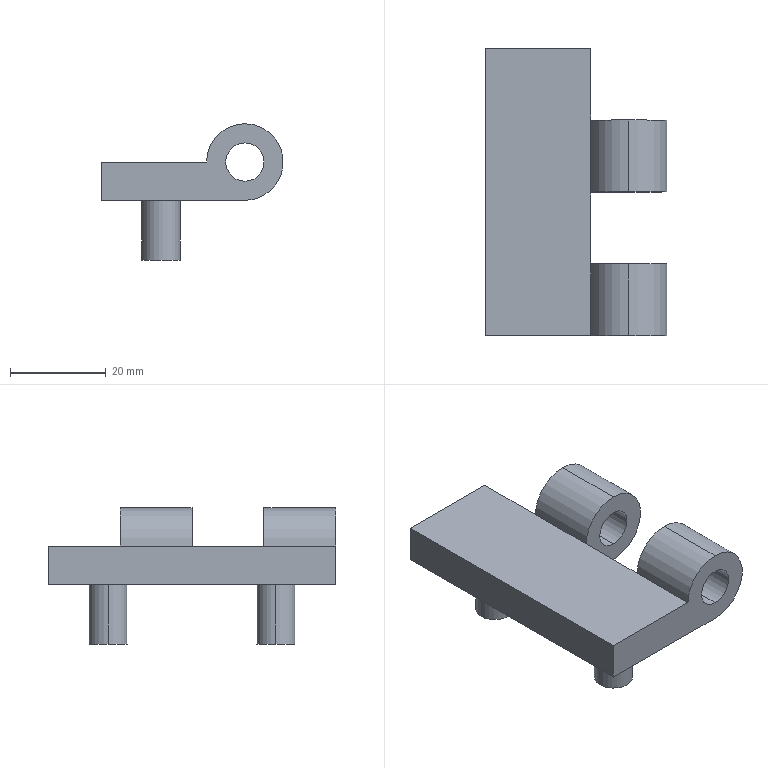Component | SolidWorks | DoorHinge2-2 | 1 solid | 24 faces | box 38 x 60 x 28.5 mm | volume 16753 mm3 | cylinder 12 | plane 12 | commonest cylinder face diameters 8 x8 16 x4
build123d program:
from build123d import *

# Parameters (mm, degrees)
SKETCH2_R           = 8
BOSS_EXTRUDE2_DEPTH = 60
SKETCH3_R           = 4
BOSS_EXTRUDE3_DEPTH = 12.5
SKETCH4_R           = 4
CUT_EXTRUDE1_DEPTH  = 71.144
SKETCH6_W           = 16
SKETCH6_H           = 15
CUT_EXTRUDE3_DEPTH  = 58


with BuildPart() as part:
    # Sketch2 → Boss-Extrude2 (new body)
    with BuildSketch(Plane(origin=(0, 0, 0), x_dir=(1, 0, 0), z_dir=(0, 1, 0))):
        Circle(SKETCH2_R)
        with BuildLine():
            ThreePointArc((8, 0), (5.657, -5.657), (0, -8))
            Line((0, -8), (30, -8))
            Line((30, -8), (30, 0))
            Line((30, 0), (8, 0))
        make_face()
    extrude(amount=BOSS_EXTRUDE2_DEPTH)

    # Sketch3 → Boss-Extrude3 (add)
    with BuildSketch(Plane.XY.offset(8)):
        with Locations(Location((17.5, 47.5, 0), (0, 0, 180))):
            Circle(SKETCH3_R)
        with Locations(Location((17.5, 12.5, 0), (0, 0, 180))):
            Circle(SKETCH3_R)
    extrude(amount=BOSS_EXTRUDE3_DEPTH)

    # Sketch4 → Cut-Extrude1 (cut, through all)
    with BuildSketch(Plane(origin=(0, 60, 0), x_dir=(1, 0, 0), z_dir=(0, 1, 0))):
        with Locations(Location((0, 0, 0), (0, 0, 270))):
            Circle(SKETCH4_R)
    extrude(amount=-CUT_EXTRUDE1_DEPTH, mode=Mode.SUBTRACT)

    # Sketch6 → Cut-Extrude3 (cut)
    with BuildSketch(Plane.XY.offset(8)):
        with Locations((0, 52.5)):
            Rectangle(SKETCH6_W, SKETCH6_H)
        with Locations((0, 22.5)):
            Rectangle(SKETCH6_W, SKETCH6_H)
    extrude(amount=-CUT_EXTRUDE3_DEPTH, mode=Mode.SUBTRACT)


solid = part.part

# Placed as in the assembly
solid = solid.moved(Location((2175.473, 210.46, 1245.107), (-180, 0, 180)))
STEP:
#1=CARTESIAN_POINT('',(85.649,9.467,48.862));
#2=VERTEX_POINT('',#1);
#3=CARTESIAN_POINT('',(85.649,9.467,49.177));
#4=VERTEX_POINT('',#3);
#5=CARTESIAN_POINT('',(85.649,9.467,49.02));
#6=DIRECTION('',(0.,-1.,0.));
#7=DIRECTION('',(0.,0.,-1.));
#8=AXIS2_PLACEMENT_3D('',#5,#6,#7);
#9=CIRCLE('',#8,0.1575);
#10=EDGE_CURVE('',#2,#4,#9,.T.);
#11=ORIENTED_EDGE('',*,*,#10,.T.);
#12=CARTESIAN_POINT('',(85.649,10.057,49.177));
#13=VERTEX_POINT('',#12);
#14=CARTESIAN_POINT('',(85.649,8.286,49.177));
#15=DIRECTION('',(-0.,1.,-0.));
#16=VECTOR('',#15,39.37);
#17=LINE('',#14,#16);
#18=EDGE_CURVE('',#4,#13,#17,.T.);
#19=ORIENTED_EDGE('',*,*,#18,.T.);
#20=CARTESIAN_POINT('',(85.649,10.057,48.862));
#21=VERTEX_POINT('',#20);
#22=CARTESIAN_POINT('',(85.649,10.057,49.02));
#23=DIRECTION('',(-0.,1.,-0.));
#24=DIRECTION('',(0.,0.,1.));
#25=AXIS2_PLACEMENT_3D('',#22,#23,#24);
#26=CIRCLE('',#25,0.1575);
#27=EDGE_CURVE('',#13,#21,#26,.T.);
#28=ORIENTED_EDGE('',*,*,#27,.T.);
#29=CARTESIAN_POINT('',(85.649,8.286,48.862));
#30=DIRECTION('',(-0.,1.,-0.));
#31=VECTOR('',#30,39.37);
#32=LINE('',#29,#31);
#33=EDGE_CURVE('',#2,#21,#32,.T.);
#34=ORIENTED_EDGE('',*,*,#33,.F.);
#35=EDGE_LOOP('',(#11,#19,#28,#34));
#36=FACE_OUTER_BOUND('',#35,.T.);
#37=CARTESIAN_POINT('',(85.649,8.286,49.02));
#38=DIRECTION('',(-0.,1.,-0.));
#39=DIRECTION('',(0.,0.,-1.));
#40=AXIS2_PLACEMENT_3D('',#37,#38,#39);
#41=CYLINDRICAL_SURFACE('',#40,0.1575);
#42=ADVANCED_FACE('',(#36),#41,.F.);
#43=CARTESIAN_POINT('',(84.802,8.778,48.213));
#44=VERTEX_POINT('',#43);
#45=CARTESIAN_POINT('',(85.117,8.778,48.213));
#46=VERTEX_POINT('',#45);
#47=CARTESIAN_POINT('',(84.96,8.778,48.213));
#48=DIRECTION('',(0.,0.,-1.));
#49=DIRECTION('',(-1.,0.,0.));
#50=AXIS2_PLACEMENT_3D('',#47,#48,#49);
#51=CIRCLE('',#50,0.1575);
#52=EDGE_CURVE('',#44,#46,#51,.T.);
#53=ORIENTED_EDGE('',*,*,#52,.F.);
#54=CARTESIAN_POINT('',(84.802,8.778,48.705));
#55=VERTEX_POINT('',#54);
#56=CARTESIAN_POINT('',(84.802,8.778,48.213));
#57=DIRECTION('',(0.,-0.,1.));
#58=VECTOR('',#57,39.37);
#59=LINE('',#56,#58);
#60=EDGE_CURVE('',#44,#55,#59,.T.);
#61=ORIENTED_EDGE('',*,*,#60,.T.);
#62=CARTESIAN_POINT('',(85.117,8.778,48.705));
#63=VERTEX_POINT('',#62);
#64=CARTESIAN_POINT('',(84.96,8.778,48.705));
#65=DIRECTION('',(0.,0.,-1.));
#66=DIRECTION('',(1.,0.,0.));
#67=AXIS2_PLACEMENT_3D('',#64,#65,#66);
#68=CIRCLE('',#67,0.1575);
#69=EDGE_CURVE('',#55,#63,#68,.T.);
#70=ORIENTED_EDGE('',*,*,#69,.T.);
#71=CARTESIAN_POINT('',(85.117,8.778,48.213));
#72=DIRECTION('',(0.,-0.,1.));
#73=VECTOR('',#72,39.37);
#74=LINE('',#71,#73);
#75=EDGE_CURVE('',#46,#63,#74,.T.);
#76=ORIENTED_EDGE('',*,*,#75,.F.);
#77=EDGE_LOOP('',(#53,#61,#70,#76));
#78=FACE_OUTER_BOUND('',#77,.T.);
#79=CARTESIAN_POINT('',(84.96,8.778,48.213));
#80=DIRECTION('',(0.,-0.,1.));
#81=DIRECTION('',(1.,0.,0.));
#82=AXIS2_PLACEMENT_3D('',#79,#80,#81);
#83=CYLINDRICAL_SURFACE('',#82,0.1575);
#84=ADVANCED_FACE('',(#78),#83,.T.);
#85=CARTESIAN_POINT('',(84.802,10.156,48.213));
#86=VERTEX_POINT('',#85);
#87=CARTESIAN_POINT('',(85.117,10.156,48.213));
#88=VERTEX_POINT('',#87);
#89=CARTESIAN_POINT('',(84.96,10.156,48.213));
#90=DIRECTION('',(0.,0.,-1.));
#91=DIRECTION('',(-1.,0.,0.));
#92=AXIS2_PLACEMENT_3D('',#89,#90,#91);
#93=CIRCLE('',#92,0.1575);
#94=EDGE_CURVE('',#86,#88,#93,.T.);
#95=ORIENTED_EDGE('',*,*,#94,.F.);
#96=CARTESIAN_POINT('',(84.802,10.156,48.705));
#97=VERTEX_POINT('',#96);
#98=CARTESIAN_POINT('',(84.802,10.156,48.213));
#99=DIRECTION('',(0.,-0.,1.));
#100=VECTOR('',#99,39.37);
#101=LINE('',#98,#100);
#102=EDGE_CURVE('',#86,#97,#101,.T.);
#103=ORIENTED_EDGE('',*,*,#102,.T.);
#104=CARTESIAN_POINT('',(85.117,10.156,48.705));
#105=VERTEX_POINT('',#104);
#106=CARTESIAN_POINT('',(84.96,10.156,48.705));
#107=DIRECTION('',(0.,0.,-1.));
#108=DIRECTION('',(1.,0.,0.));
#109=AXIS2_PLACEMENT_3D('',#106,#107,#108);
#110=CIRCLE('',#109,0.1575);
#111=EDGE_CURVE('',#97,#105,#110,.T.);
#112=ORIENTED_EDGE('',*,*,#111,.T.);
#113=CARTESIAN_POINT('',(85.117,10.156,48.213));
#114=DIRECTION('',(0.,-0.,1.));
#115=VECTOR('',#114,39.37);
#116=LINE('',#113,#115);
#117=EDGE_CURVE('',#88,#105,#116,.T.);
#118=ORIENTED_EDGE('',*,*,#117,.F.);
#119=EDGE_LOOP('',(#95,#103,#112,#118));
#120=FACE_OUTER_BOUND('',#119,.T.);
#121=CARTESIAN_POINT('',(84.96,10.156,48.213));
#122=DIRECTION('',(0.,-0.,1.));
#123=DIRECTION('',(1.,0.,0.));
#124=AXIS2_PLACEMENT_3D('',#121,#122,#123);
#125=CYLINDRICAL_SURFACE('',#124,0.1575);
#126=ADVANCED_FACE('',(#120),#125,.T.);
#127=CARTESIAN_POINT('',(85.649,10.057,48.705));
#128=VERTEX_POINT('',#127);
#129=CARTESIAN_POINT('',(85.649,10.057,49.335));
#130=VERTEX_POINT('',#129);
#131=CARTESIAN_POINT('',(85.649,10.057,49.02));
#132=DIRECTION('',(0.,-1.,0.));
#133=DIRECTION('',(0.,0.,1.));
#134=AXIS2_PLACEMENT_3D('',#131,#132,#133);
#135=CIRCLE('',#134,0.315);
#136=EDGE_CURVE('',#128,#130,#135,.T.);
#137=ORIENTED_EDGE('',*,*,#136,.T.);
#138=CARTESIAN_POINT('',(85.649,9.467,49.335));
#139=VERTEX_POINT('',#138);
#140=CARTESIAN_POINT('',(85.649,10.648,49.335));
#141=DIRECTION('',(0.,-1.,0.));
#142=VECTOR('',#141,39.37);
#143=LINE('',#140,#142);
#144=EDGE_CURVE('',#130,#139,#143,.T.);
#145=ORIENTED_EDGE('',*,*,#144,.T.);
#146=CARTESIAN_POINT('',(85.649,9.467,48.705));
#147=VERTEX_POINT('',#146);
#148=CARTESIAN_POINT('',(85.649,9.467,49.02));
#149=DIRECTION('',(-0.,1.,-0.));
#150=DIRECTION('',(0.,0.,-1.));
#151=AXIS2_PLACEMENT_3D('',#148,#149,#150);
#152=CIRCLE('',#151,0.315);
#153=EDGE_CURVE('',#139,#147,#152,.T.);
#154=ORIENTED_EDGE('',*,*,#153,.T.);
#155=CARTESIAN_POINT('',(85.649,10.648,48.705));
#156=DIRECTION('',(0.,-1.,0.));
#157=VECTOR('',#156,39.37);
#158=LINE('',#155,#157);
#159=EDGE_CURVE('',#128,#147,#158,.T.);
#160=ORIENTED_EDGE('',*,*,#159,.F.);
#161=EDGE_LOOP('',(#137,#145,#154,#160));
#162=FACE_OUTER_BOUND('',#161,.T.);
#163=CARTESIAN_POINT('',(85.649,10.648,49.02));
#164=DIRECTION('',(0.,-1.,0.));
#165=DIRECTION('',(0.,0.,1.));
#166=AXIS2_PLACEMENT_3D('',#163,#164,#165);
#167=CYLINDRICAL_SURFACE('',#166,0.315);
#168=ADVANCED_FACE('',(#162),#167,.T.);
#169=CARTESIAN_POINT('',(85.649,8.286,49.177));
#170=VERTEX_POINT('',#169);
#171=CARTESIAN_POINT('',(85.649,8.286,48.862));
#172=VERTEX_POINT('',#171);
#173=CARTESIAN_POINT('',(85.649,8.286,49.02));
#174=DIRECTION('',(-0.,1.,-0.));
#175=DIRECTION('',(0.,0.,-1.));
#176=AXIS2_PLACEMENT_3D('',#173,#174,#175);
#177=CIRCLE('',#176,0.1575);
#178=EDGE_CURVE('',#170,#172,#177,.T.);
#179=ORIENTED_EDGE('',*,*,#178,.F.);
#180=CARTESIAN_POINT('',(85.649,8.876,49.177));
#181=VERTEX_POINT('',#180);
#182=CARTESIAN_POINT('',(85.649,8.286,49.177));
#183=DIRECTION('',(-0.,1.,-0.));
#184=VECTOR('',#183,39.37);
#185=LINE('',#182,#184);
#186=EDGE_CURVE('',#170,#181,#185,.T.);
#187=ORIENTED_EDGE('',*,*,#186,.T.);
#188=CARTESIAN_POINT('',(85.649,8.876,48.862));
#189=VERTEX_POINT('',#188);
#190=CARTESIAN_POINT('',(85.649,8.876,49.02));
#191=DIRECTION('',(0.,1.,-0.));
#192=DIRECTION('',(-1.,0.,0.));
#193=AXIS2_PLACEMENT_3D('',#190,#191,#192);
#194=CIRCLE('',#193,0.1575);
#195=EDGE_CURVE('',#181,#189,#194,.T.);
#196=ORIENTED_EDGE('',*,*,#195,.T.);
#197=CARTESIAN_POINT('',(85.649,8.286,48.862));
#198=DIRECTION('',(-0.,1.,-0.));
#199=VECTOR('',#198,39.37);
#200=LINE('',#197,#199);
#201=EDGE_CURVE('',#172,#189,#200,.T.);
#202=ORIENTED_EDGE('',*,*,#201,.F.);
#203=EDGE_LOOP('',(#179,#187,#196,#202));
#204=FACE_OUTER_BOUND('',#203,.T.);
#205=CARTESIAN_POINT('',(85.649,8.286,49.02));
#206=DIRECTION('',(-0.,1.,-0.));
#207=DIRECTION('',(0.,0.,-1.));
#208=AXIS2_PLACEMENT_3D('',#205,#206,#207);
#209=CYLINDRICAL_SURFACE('',#208,0.1575);
#210=ADVANCED_FACE('',(#204),#209,.F.);
#211=CARTESIAN_POINT('',(85.649,8.876,48.705));
#212=VERTEX_POINT('',#211);
#213=CARTESIAN_POINT('',(85.649,8.876,49.335));
#214=VERTEX_POINT('',#213);
#215=CARTESIAN_POINT('',(85.649,8.876,49.02));
#216=DIRECTION('',(-0.,-1.,0.));
#217=DIRECTION('',(-1.,0.,0.));
#218=AXIS2_PLACEMENT_3D('',#215,#216,#217);
#219=CIRCLE('',#218,0.315);
#220=EDGE_CURVE('',#212,#214,#219,.T.);
#221=ORIENTED_EDGE('',*,*,#220,.T.);
#222=CARTESIAN_POINT('',(85.649,8.286,49.335));
#223=VERTEX_POINT('',#222);
#224=CARTESIAN_POINT('',(85.649,10.648,49.335));
#225=DIRECTION('',(0.,-1.,0.));
#226=VECTOR('',#225,39.37);
#227=LINE('',#224,#226);
#228=EDGE_CURVE('',#214,#223,#227,.T.);
#229=ORIENTED_EDGE('',*,*,#228,.T.);
#230=CARTESIAN_POINT('',(85.649,8.286,48.705));
#231=VERTEX_POINT('',#230);
#232=CARTESIAN_POINT('',(85.649,8.286,49.02));
#233=DIRECTION('',(-0.,1.,-0.));
#234=DIRECTION('',(0.,0.,-1.));
#235=AXIS2_PLACEMENT_3D('',#232,#233,#234);
#236=CIRCLE('',#235,0.315);
#237=EDGE_CURVE('',#223,#231,#236,.T.);
#238=ORIENTED_EDGE('',*,*,#237,.T.);
#239=CARTESIAN_POINT('',(85.649,10.648,48.705));
#240=DIRECTION('',(0.,-1.,0.));
#241=VECTOR('',#240,39.37);
#242=LINE('',#239,#241);
#243=EDGE_CURVE('',#212,#231,#242,.T.);
#244=ORIENTED_EDGE('',*,*,#243,.F.);
#245=EDGE_LOOP('',(#221,#229,#238,#244));
#246=FACE_OUTER_BOUND('',#245,.T.);
#247=CARTESIAN_POINT('',(85.649,10.648,49.02));
#248=DIRECTION('',(0.,-1.,0.));
#249=DIRECTION('',(0.,0.,1.));
#250=AXIS2_PLACEMENT_3D('',#247,#248,#249);
#251=CYLINDRICAL_SURFACE('',#250,0.315);
#252=ADVANCED_FACE('',(#246),#251,.T.);
#253=ORIENTED_EDGE('',*,*,#228,.F.);
#254=CARTESIAN_POINT('',(85.334,8.876,49.02));
#255=VERTEX_POINT('',#254);
#256=CARTESIAN_POINT('',(85.649,8.876,49.02));
#257=DIRECTION('',(-0.,-1.,0.));
#258=DIRECTION('',(-1.,0.,0.));
#259=AXIS2_PLACEMENT_3D('',#256,#257,#258);
#260=CIRCLE('',#259,0.315);
#261=EDGE_CURVE('',#214,#255,#260,.T.);
#262=ORIENTED_EDGE('',*,*,#261,.T.);
#263=CARTESIAN_POINT('',(85.334,8.286,49.02));
#264=VERTEX_POINT('',#263);
#265=CARTESIAN_POINT('',(85.334,10.648,49.02));
#266=DIRECTION('',(0.,-1.,0.));
#267=VECTOR('',#266,39.37);
#268=LINE('',#265,#267);
#269=EDGE_CURVE('',#255,#264,#268,.T.);
#270=ORIENTED_EDGE('',*,*,#269,.T.);
#271=CARTESIAN_POINT('',(85.649,8.286,49.02));
#272=DIRECTION('',(-0.,1.,-0.));
#273=DIRECTION('',(0.,0.,-1.));
#274=AXIS2_PLACEMENT_3D('',#271,#272,#273);
#275=CIRCLE('',#274,0.315);
#276=EDGE_CURVE('',#264,#223,#275,.T.);
#277=ORIENTED_EDGE('',*,*,#276,.T.);
#278=EDGE_LOOP('',(#253,#262,#270,#277));
#279=FACE_OUTER_BOUND('',#278,.T.);
#280=CARTESIAN_POINT('',(85.649,10.648,49.02));
#281=DIRECTION('',(0.,-1.,0.));
#282=DIRECTION('',(0.,0.,1.));
#283=AXIS2_PLACEMENT_3D('',#280,#281,#282);
#284=CYLINDRICAL_SURFACE('',#283,0.315);
#285=ADVANCED_FACE('',(#279),#284,.T.);
#286=ORIENTED_EDGE('',*,*,#186,.F.);
#287=CARTESIAN_POINT('',(85.649,8.286,49.02));
#288=DIRECTION('',(-0.,1.,-0.));
#289=DIRECTION('',(0.,0.,-1.));
#290=AXIS2_PLACEMENT_3D('',#287,#288,#289);
#291=CIRCLE('',#290,0.1575);
#292=EDGE_CURVE('',#172,#170,#291,.T.);
#293=ORIENTED_EDGE('',*,*,#292,.F.);
#294=ORIENTED_EDGE('',*,*,#201,.T.);
#295=CARTESIAN_POINT('',(85.649,8.876,49.02));
#296=DIRECTION('',(0.,1.,-0.));
#297=DIRECTION('',(-1.,0.,0.));
#298=AXIS2_PLACEMENT_3D('',#295,#296,#297);
#299=CIRCLE('',#298,0.1575);
#300=EDGE_CURVE('',#189,#181,#299,.T.);
#301=ORIENTED_EDGE('',*,*,#300,.T.);
#302=EDGE_LOOP('',(#286,#293,#294,#301));
#303=FACE_OUTER_BOUND('',#302,.T.);
#304=CARTESIAN_POINT('',(85.649,8.286,49.02));
#305=DIRECTION('',(-0.,1.,-0.));
#306=DIRECTION('',(0.,0.,-1.));
#307=AXIS2_PLACEMENT_3D('',#304,#305,#306);
#308=CYLINDRICAL_SURFACE('',#307,0.1575);
#309=ADVANCED_FACE('',(#303),#308,.F.);
#310=CARTESIAN_POINT('',(84.96,10.156,48.705));
#311=DIRECTION('',(0.,0.,-1.));
#312=DIRECTION('',(1.,0.,0.));
#313=AXIS2_PLACEMENT_3D('',#310,#311,#312);
#314=CIRCLE('',#313,0.1575);
#315=EDGE_CURVE('',#105,#97,#314,.T.);
#316=ORIENTED_EDGE('',*,*,#315,.F.);
#317=ORIENTED_EDGE('',*,*,#111,.F.);
#318=EDGE_LOOP('',(#316,#317));
#319=FACE_BOUND('',#318,.T.);
#320=CARTESIAN_POINT('',(85.334,8.876,48.705));
#321=VERTEX_POINT('',#320);
#322=CARTESIAN_POINT('',(85.334,9.467,48.705));
#323=VERTEX_POINT('',#322);
#324=CARTESIAN_POINT('',(85.334,8.876,48.705));
#325=DIRECTION('',(0.,1.,-0.));
#326=VECTOR('',#325,39.37);
#327=LINE('',#324,#326);
#328=EDGE_CURVE('',#321,#323,#327,.T.);
#329=ORIENTED_EDGE('',*,*,#328,.F.);
#330=CARTESIAN_POINT('',(85.334,8.876,48.705));
#331=DIRECTION('',(-1.,0.,-0.));
#332=VECTOR('',#331,39.37);
#333=LINE('',#330,#332);
#334=EDGE_CURVE('',#212,#321,#333,.T.);
#335=ORIENTED_EDGE('',*,*,#334,.F.);
#336=ORIENTED_EDGE('',*,*,#243,.T.);
#337=CARTESIAN_POINT('',(84.467,8.286,48.705));
#338=VERTEX_POINT('',#337);
#339=CARTESIAN_POINT('',(86.484,8.286,48.705));
#340=DIRECTION('',(-1.,0.,0.));
#341=VECTOR('',#340,39.37);
#342=LINE('',#339,#341);
#343=EDGE_CURVE('',#231,#338,#342,.T.);
#344=ORIENTED_EDGE('',*,*,#343,.T.);
#345=CARTESIAN_POINT('',(84.467,10.648,48.705));
#346=VERTEX_POINT('',#345);
#347=CARTESIAN_POINT('',(84.467,10.648,48.705));
#348=DIRECTION('',(0.,-1.,0.));
#349=VECTOR('',#348,39.37);
#350=LINE('',#347,#349);
#351=EDGE_CURVE('',#346,#338,#350,.T.);
#352=ORIENTED_EDGE('',*,*,#351,.F.);
#353=CARTESIAN_POINT('',(85.334,10.648,48.705));
#354=VERTEX_POINT('',#353);
#355=CARTESIAN_POINT('',(86.484,10.648,48.705));
#356=DIRECTION('',(-1.,0.,0.));
#357=VECTOR('',#356,39.37);
#358=LINE('',#355,#357);
#359=EDGE_CURVE('',#354,#346,#358,.T.);
#360=ORIENTED_EDGE('',*,*,#359,.F.);
#361=CARTESIAN_POINT('',(85.334,10.057,48.705));
#362=VERTEX_POINT('',#361);
#363=CARTESIAN_POINT('',(85.334,10.057,48.705));
#364=DIRECTION('',(0.,1.,-0.));
#365=VECTOR('',#364,39.37);
#366=LINE('',#363,#365);
#367=EDGE_CURVE('',#362,#354,#366,.T.);
#368=ORIENTED_EDGE('',*,*,#367,.F.);
#369=CARTESIAN_POINT('',(85.334,10.057,48.705));
#370=DIRECTION('',(-1.,0.,0.));
#371=VECTOR('',#370,39.37);
#372=LINE('',#369,#371);
#373=EDGE_CURVE('',#128,#362,#372,.T.);
#374=ORIENTED_EDGE('',*,*,#373,.F.);
#375=ORIENTED_EDGE('',*,*,#159,.T.);
#376=CARTESIAN_POINT('',(85.334,9.467,48.705));
#377=DIRECTION('',(1.,0.,0.));
#378=VECTOR('',#377,39.37);
#379=LINE('',#376,#378);
#380=EDGE_CURVE('',#323,#147,#379,.T.);
#381=ORIENTED_EDGE('',*,*,#380,.F.);
#382=EDGE_LOOP('',(#329,#335,#336,#344,#352,#360,#368,#374,#375,#381));
#383=FACE_OUTER_BOUND('',#382,.T.);
#384=CARTESIAN_POINT('',(84.96,8.778,48.705));
#385=DIRECTION('',(0.,0.,-1.));
#386=DIRECTION('',(1.,0.,0.));
#387=AXIS2_PLACEMENT_3D('',#384,#385,#386);
#388=CIRCLE('',#387,0.1575);
#389=EDGE_CURVE('',#63,#55,#388,.T.);
#390=ORIENTED_EDGE('',*,*,#389,.F.);
#391=ORIENTED_EDGE('',*,*,#69,.F.);
#392=EDGE_LOOP('',(#390,#391));
#393=FACE_BOUND('',#392,.T.);
#394=CARTESIAN_POINT('',(86.484,10.648,48.705));
#395=DIRECTION('',(0.,-0.,1.));
#396=DIRECTION('',(1.,0.,0.));
#397=AXIS2_PLACEMENT_3D('',#394,#395,#396);
#398=PLANE('',#397);
#399=ADVANCED_FACE('',(#319,#383,#393),#398,.F.);
#400=ORIENTED_EDGE('',*,*,#144,.F.);
#401=CARTESIAN_POINT('',(85.334,10.057,49.02));
#402=VERTEX_POINT('',#401);
#403=CARTESIAN_POINT('',(85.649,10.057,49.02));
#404=DIRECTION('',(0.,-1.,0.));
#405=DIRECTION('',(0.,0.,1.));
#406=AXIS2_PLACEMENT_3D('',#403,#404,#405);
#407=CIRCLE('',#406,0.315);
#408=EDGE_CURVE('',#130,#402,#407,.T.);
#409=ORIENTED_EDGE('',*,*,#408,.T.);
#410=CARTESIAN_POINT('',(85.334,9.467,49.02));
#411=VERTEX_POINT('',#410);
#412=CARTESIAN_POINT('',(85.334,10.648,49.02));
#413=DIRECTION('',(0.,-1.,0.));
#414=VECTOR('',#413,39.37);
#415=LINE('',#412,#414);
#416=EDGE_CURVE('',#402,#411,#415,.T.);
#417=ORIENTED_EDGE('',*,*,#416,.T.);
#418=CARTESIAN_POINT('',(85.649,9.467,49.02));
#419=DIRECTION('',(-0.,1.,-0.));
#420=DIRECTION('',(0.,0.,-1.));
#421=AXIS2_PLACEMENT_3D('',#418,#419,#420);
#422=CIRCLE('',#421,0.315);
#423=EDGE_CURVE('',#411,#139,#422,.T.);
#424=ORIENTED_EDGE('',*,*,#423,.T.);
#425=EDGE_LOOP('',(#400,#409,#417,#424));
#426=FACE_OUTER_BOUND('',#425,.T.);
#427=CARTESIAN_POINT('',(85.649,10.648,49.02));
#428=DIRECTION('',(0.,-1.,0.));
#429=DIRECTION('',(0.,0.,1.));
#430=AXIS2_PLACEMENT_3D('',#427,#428,#429);
#431=CYLINDRICAL_SURFACE('',#430,0.315);
#432=ADVANCED_FACE('',(#426),#431,.T.);
#433=CARTESIAN_POINT('',(84.467,8.286,49.02));
#434=VERTEX_POINT('',#433);
#435=CARTESIAN_POINT('',(84.467,8.286,49.02));
#436=DIRECTION('',(0.,-0.,1.));
#437=VECTOR('',#436,39.37);
#438=LINE('',#435,#437);
#439=EDGE_CURVE('',#338,#434,#438,.T.);
#440=ORIENTED_EDGE('',*,*,#439,.T.);
#441=CARTESIAN_POINT('',(84.467,10.648,49.02));
#442=VERTEX_POINT('',#441);
#443=CARTESIAN_POINT('',(84.467,10.648,49.02));
#444=DIRECTION('',(0.,-1.,0.));
#445=VECTOR('',#444,39.37);
#446=LINE('',#443,#445);
#447=EDGE_CURVE('',#442,#434,#446,.T.);
#448=ORIENTED_EDGE('',*,*,#447,.F.);
#449=CARTESIAN_POINT('',(84.467,10.648,49.02));
#450=DIRECTION('',(0.,-0.,1.));
#451=VECTOR('',#450,39.37);
#452=LINE('',#449,#451);
#453=EDGE_CURVE('',#346,#442,#452,.T.);
#454=ORIENTED_EDGE('',*,*,#453,.F.);
#455=ORIENTED_EDGE('',*,*,#351,.T.);
#456=EDGE_LOOP('',(#440,#448,#454,#455));
#457=FACE_OUTER_BOUND('',#456,.T.);
#458=CARTESIAN_POINT('',(84.467,10.648,49.02));
#459=DIRECTION('',(1.,0.,0.));
#460=DIRECTION('',(0.,0.,-1.));
#461=AXIS2_PLACEMENT_3D('',#458,#459,#460);
#462=PLANE('',#461);
#463=ADVANCED_FACE('',(#457),#462,.F.);
#464=CARTESIAN_POINT('',(86.484,8.286,49.02));
#465=DIRECTION('',(1.,-0.,0.));
#466=VECTOR('',#465,39.37);
#467=LINE('',#464,#466);
#468=EDGE_CURVE('',#434,#264,#467,.T.);
#469=ORIENTED_EDGE('',*,*,#468,.T.);
#470=ORIENTED_EDGE('',*,*,#269,.F.);
#471=CARTESIAN_POINT('',(85.334,10.648,49.02));
#472=DIRECTION('',(0.,-1.,0.));
#473=VECTOR('',#472,39.37);
#474=LINE('',#471,#473);
#475=EDGE_CURVE('',#411,#255,#474,.T.);
#476=ORIENTED_EDGE('',*,*,#475,.F.);
#477=ORIENTED_EDGE('',*,*,#416,.F.);
#478=CARTESIAN_POINT('',(85.334,10.648,49.02));
#479=VERTEX_POINT('',#478);
#480=CARTESIAN_POINT('',(85.334,10.648,49.02));
#481=DIRECTION('',(0.,-1.,0.));
#482=VECTOR('',#481,39.37);
#483=LINE('',#480,#482);
#484=EDGE_CURVE('',#479,#402,#483,.T.);
#485=ORIENTED_EDGE('',*,*,#484,.F.);
#486=CARTESIAN_POINT('',(86.484,10.648,49.02));
#487=DIRECTION('',(1.,-0.,0.));
#488=VECTOR('',#487,39.37);
#489=LINE('',#486,#488);
#490=EDGE_CURVE('',#442,#479,#489,.T.);
#491=ORIENTED_EDGE('',*,*,#490,.F.);
#492=ORIENTED_EDGE('',*,*,#447,.T.);
#493=EDGE_LOOP('',(#469,#470,#476,#477,#485,#491,#492));
#494=FACE_OUTER_BOUND('',#493,.T.);
#495=CARTESIAN_POINT('',(86.484,10.648,49.02));
#496=DIRECTION('',(0.,0.,-1.));
#497=DIRECTION('',(-1.,0.,-0.));
#498=AXIS2_PLACEMENT_3D('',#495,#496,#497);
#499=PLANE('',#498);
#500=ADVANCED_FACE('',(#494),#499,.F.);
#501=CARTESIAN_POINT('',(85.334,10.648,50.988));
#502=DIRECTION('',(0.,0.,-1.));
#503=VECTOR('',#502,39.37);
#504=LINE('',#501,#503);
#505=EDGE_CURVE('',#479,#354,#504,.T.);
#506=ORIENTED_EDGE('',*,*,#505,.T.);
#507=ORIENTED_EDGE('',*,*,#359,.T.);
#508=ORIENTED_EDGE('',*,*,#453,.T.);
#509=ORIENTED_EDGE('',*,*,#490,.T.);
#510=EDGE_LOOP('',(#506,#507,#508,#509));
#511=FACE_OUTER_BOUND('',#510,.T.);
#512=CARTESIAN_POINT('',(86.484,10.648,49.02));
#513=DIRECTION('',(-0.,1.,0.));
#514=DIRECTION('',(0.,0.,-1.));
#515=AXIS2_PLACEMENT_3D('',#512,#513,#514);
#516=PLANE('',#515);
#517=ADVANCED_FACE('',(#511),#516,.T.);
#518=ORIENTED_EDGE('',*,*,#292,.T.);
#519=ORIENTED_EDGE('',*,*,#178,.T.);
#520=EDGE_LOOP('',(#518,#519));
#521=FACE_BOUND('',#520,.T.);
#522=ORIENTED_EDGE('',*,*,#276,.F.);
#523=ORIENTED_EDGE('',*,*,#468,.F.);
#524=ORIENTED_EDGE('',*,*,#439,.F.);
#525=ORIENTED_EDGE('',*,*,#343,.F.);
#526=ORIENTED_EDGE('',*,*,#237,.F.);
#527=EDGE_LOOP('',(#522,#523,#524,#525,#526));
#528=FACE_OUTER_BOUND('',#527,.T.);
#529=CARTESIAN_POINT('',(86.484,8.286,49.02));
#530=DIRECTION('',(-0.,1.,0.));
#531=DIRECTION('',(0.,0.,-1.));
#532=AXIS2_PLACEMENT_3D('',#529,#530,#531);
#533=PLANE('',#532);
#534=ADVANCED_FACE('',(#521,#528),#533,.F.);
#535=ORIENTED_EDGE('',*,*,#102,.F.);
#536=CARTESIAN_POINT('',(84.96,10.156,48.213));
#537=DIRECTION('',(0.,0.,-1.));
#538=DIRECTION('',(-1.,0.,0.));
#539=AXIS2_PLACEMENT_3D('',#536,#537,#538);
#540=CIRCLE('',#539,0.1575);
#541=EDGE_CURVE('',#88,#86,#540,.T.);
#542=ORIENTED_EDGE('',*,*,#541,.F.);
#543=ORIENTED_EDGE('',*,*,#117,.T.);
#544=ORIENTED_EDGE('',*,*,#315,.T.);
#545=EDGE_LOOP('',(#535,#542,#543,#544));
#546=FACE_OUTER_BOUND('',#545,.T.);
#547=CARTESIAN_POINT('',(84.96,10.156,48.213));
#548=DIRECTION('',(0.,-0.,1.));
#549=DIRECTION('',(1.,0.,0.));
#550=AXIS2_PLACEMENT_3D('',#547,#548,#549);
#551=CYLINDRICAL_SURFACE('',#550,0.1575);
#552=ADVANCED_FACE('',(#546),#551,.T.);
#553=ORIENTED_EDGE('',*,*,#541,.T.);
#554=ORIENTED_EDGE('',*,*,#94,.T.);
#555=EDGE_LOOP('',(#553,#554));
#556=FACE_OUTER_BOUND('',#555,.T.);
#557=CARTESIAN_POINT('',(84.96,10.156,48.213));
#558=DIRECTION('',(0.,0.,-1.));
#559=DIRECTION('',(-1.,0.,0.));
#560=AXIS2_PLACEMENT_3D('',#557,#558,#559);
#561=PLANE('',#560);
#562=ADVANCED_FACE('',(#556),#561,.T.);
#563=ORIENTED_EDGE('',*,*,#60,.F.);
#564=CARTESIAN_POINT('',(84.96,8.778,48.213));
#565=DIRECTION('',(0.,0.,-1.));
#566=DIRECTION('',(-1.,0.,0.));
#567=AXIS2_PLACEMENT_3D('',#564,#565,#566);
#568=CIRCLE('',#567,0.1575);
#569=EDGE_CURVE('',#46,#44,#568,.T.);
#570=ORIENTED_EDGE('',*,*,#569,.F.);
#571=ORIENTED_EDGE('',*,*,#75,.T.);
#572=ORIENTED_EDGE('',*,*,#389,.T.);
#573=EDGE_LOOP('',(#563,#570,#571,#572));
#574=FACE_OUTER_BOUND('',#573,.T.);
#575=CARTESIAN_POINT('',(84.96,8.778,48.213));
#576=DIRECTION('',(0.,-0.,1.));
#577=DIRECTION('',(1.,0.,0.));
#578=AXIS2_PLACEMENT_3D('',#575,#576,#577);
#579=CYLINDRICAL_SURFACE('',#578,0.1575);
#580=ADVANCED_FACE('',(#574),#579,.T.);
#581=ORIENTED_EDGE('',*,*,#569,.T.);
#582=ORIENTED_EDGE('',*,*,#52,.T.);
#583=EDGE_LOOP('',(#581,#582));
#584=FACE_OUTER_BOUND('',#583,.T.);
#585=CARTESIAN_POINT('',(84.96,8.778,48.213));
#586=DIRECTION('',(0.,0.,-1.));
#587=DIRECTION('',(-1.,0.,0.));
#588=AXIS2_PLACEMENT_3D('',#585,#586,#587);
#589=PLANE('',#588);
#590=ADVANCED_FACE('',(#584),#589,.T.);
#591=ORIENTED_EDGE('',*,*,#18,.F.);
#592=CARTESIAN_POINT('',(85.649,9.467,49.02));
#593=DIRECTION('',(0.,-1.,0.));
#594=DIRECTION('',(0.,0.,-1.));
#595=AXIS2_PLACEMENT_3D('',#592,#593,#594);
#596=CIRCLE('',#595,0.1575);
#597=EDGE_CURVE('',#4,#2,#596,.T.);
#598=ORIENTED_EDGE('',*,*,#597,.T.);
#599=ORIENTED_EDGE('',*,*,#33,.T.);
#600=CARTESIAN_POINT('',(85.649,10.057,49.02));
#601=DIRECTION('',(-0.,1.,-0.));
#602=DIRECTION('',(0.,0.,1.));
#603=AXIS2_PLACEMENT_3D('',#600,#601,#602);
#604=CIRCLE('',#603,0.1575);
#605=EDGE_CURVE('',#21,#13,#604,.T.);
#606=ORIENTED_EDGE('',*,*,#605,.T.);
#607=EDGE_LOOP('',(#591,#598,#599,#606));
#608=FACE_OUTER_BOUND('',#607,.T.);
#609=CARTESIAN_POINT('',(85.649,8.286,49.02));
#610=DIRECTION('',(-0.,1.,-0.));
#611=DIRECTION('',(0.,0.,-1.));
#612=AXIS2_PLACEMENT_3D('',#609,#610,#611);
#613=CYLINDRICAL_SURFACE('',#612,0.1575);
#614=ADVANCED_FACE('',(#608),#613,.F.);
#615=CARTESIAN_POINT('',(85.334,10.057,50.988));
#616=DIRECTION('',(0.,0.,-1.));
#617=VECTOR('',#616,39.37);
#618=LINE('',#615,#617);
#619=EDGE_CURVE('',#402,#362,#618,.T.);
#620=ORIENTED_EDGE('',*,*,#619,.T.);
#621=ORIENTED_EDGE('',*,*,#367,.T.);
#622=ORIENTED_EDGE('',*,*,#505,.F.);
#623=ORIENTED_EDGE('',*,*,#484,.T.);
#624=EDGE_LOOP('',(#620,#621,#622,#623));
#625=FACE_OUTER_BOUND('',#624,.T.);
#626=CARTESIAN_POINT('',(85.334,10.057,50.988));
#627=DIRECTION('',(-1.,0.,-0.));
#628=DIRECTION('',(0.,1.,-0.));
#629=AXIS2_PLACEMENT_3D('',#626,#627,#628);
#630=PLANE('',#629);
#631=ADVANCED_FACE('',(#625),#630,.F.);
#632=ORIENTED_EDGE('',*,*,#605,.F.);
#633=ORIENTED_EDGE('',*,*,#27,.F.);
#634=EDGE_LOOP('',(#632,#633));
#635=FACE_BOUND('',#634,.T.);
#636=ORIENTED_EDGE('',*,*,#373,.T.);
#637=ORIENTED_EDGE('',*,*,#619,.F.);
#638=ORIENTED_EDGE('',*,*,#408,.F.);
#639=ORIENTED_EDGE('',*,*,#136,.F.);
#640=EDGE_LOOP('',(#636,#637,#638,#639));
#641=FACE_OUTER_BOUND('',#640,.T.);
#642=CARTESIAN_POINT('',(85.334,10.057,50.988));
#643=DIRECTION('',(0.,-1.,-0.));
#644=DIRECTION('',(0.,-0.,1.));
#645=AXIS2_PLACEMENT_3D('',#642,#643,#644);
#646=PLANE('',#645);
#647=ADVANCED_FACE('',(#635,#641),#646,.F.);
#648=CARTESIAN_POINT('',(85.334,8.876,50.988));
#649=DIRECTION('',(0.,0.,-1.));
#650=VECTOR('',#649,39.37);
#651=LINE('',#648,#650);
#652=EDGE_CURVE('',#255,#321,#651,.T.);
#653=ORIENTED_EDGE('',*,*,#652,.T.);
#654=ORIENTED_EDGE('',*,*,#328,.T.);
#655=CARTESIAN_POINT('',(85.334,9.467,50.988));
#656=DIRECTION('',(0.,0.,-1.));
#657=VECTOR('',#656,39.37);
#658=LINE('',#655,#657);
#659=EDGE_CURVE('',#411,#323,#658,.T.);
#660=ORIENTED_EDGE('',*,*,#659,.F.);
#661=ORIENTED_EDGE('',*,*,#475,.T.);
#662=EDGE_LOOP('',(#653,#654,#660,#661));
#663=FACE_OUTER_BOUND('',#662,.T.);
#664=CARTESIAN_POINT('',(85.334,8.876,50.988));
#665=DIRECTION('',(-1.,0.,-0.));
#666=DIRECTION('',(0.,1.,-0.));
#667=AXIS2_PLACEMENT_3D('',#664,#665,#666);
#668=PLANE('',#667);
#669=ADVANCED_FACE('',(#663),#668,.F.);
#670=ORIENTED_EDGE('',*,*,#300,.F.);
#671=ORIENTED_EDGE('',*,*,#195,.F.);
#672=EDGE_LOOP('',(#670,#671));
#673=FACE_BOUND('',#672,.T.);
#674=ORIENTED_EDGE('',*,*,#334,.T.);
#675=ORIENTED_EDGE('',*,*,#652,.F.);
#676=ORIENTED_EDGE('',*,*,#261,.F.);
#677=ORIENTED_EDGE('',*,*,#220,.F.);
#678=EDGE_LOOP('',(#674,#675,#676,#677));
#679=FACE_OUTER_BOUND('',#678,.T.);
#680=CARTESIAN_POINT('',(85.334,8.876,50.988));
#681=DIRECTION('',(-0.,-1.,0.));
#682=DIRECTION('',(-1.,0.,-0.));
#683=AXIS2_PLACEMENT_3D('',#680,#681,#682);
#684=PLANE('',#683);
#685=ADVANCED_FACE('',(#673,#679),#684,.F.);
#686=ORIENTED_EDGE('',*,*,#10,.F.);
#687=ORIENTED_EDGE('',*,*,#597,.F.);
#688=EDGE_LOOP('',(#686,#687));
#689=FACE_BOUND('',#688,.T.);
#690=ORIENTED_EDGE('',*,*,#659,.T.);
#691=ORIENTED_EDGE('',*,*,#380,.T.);
#692=ORIENTED_EDGE('',*,*,#153,.F.);
#693=ORIENTED_EDGE('',*,*,#423,.F.);
#694=EDGE_LOOP('',(#690,#691,#692,#693));
#695=FACE_OUTER_BOUND('',#694,.T.);
#696=CARTESIAN_POINT('',(85.334,9.467,50.988));
#697=DIRECTION('',(-0.,1.,0.));
#698=DIRECTION('',(0.,0.,-1.));
#699=AXIS2_PLACEMENT_3D('',#696,#697,#698);
#700=PLANE('',#699);
#701=ADVANCED_FACE('',(#689,#695),#700,.F.);
#702=CLOSED_SHELL('',(#42,#84,#126,#168,#210,#252,#285,#309,#399,#432,#463,#500,#517,#534,#552,#562,#580,#590,#614,#631,#647,#669,#685,#701));
#703=MANIFOLD_SOLID_BREP('',#702);
#704=CARTESIAN_POINT('',(0.,0.,0.));
#705=DIRECTION('',(0.,0.,1.));
#706=DIRECTION('',(1.,0.,0.));
#707=AXIS2_PLACEMENT_3D('',#704,#705,#706);
#708=(LENGTH_UNIT()NAMED_UNIT(*)SI_UNIT($,.METRE.));
#709=LENGTH_MEASURE_WITH_UNIT(LENGTH_MEASURE(0.0254),#708);
#710=DIMENSIONAL_EXPONENTS(1.,0.,0.,0.,0.,0.,0.);
#711=(CONVERSION_BASED_UNIT('',#709)LENGTH_UNIT()NAMED_UNIT(#710));
#712=UNCERTAINTY_MEASURE_WITH_UNIT(LENGTH_MEASURE(0.00001),#711,'','');
#713=(NAMED_UNIT(*)PLANE_ANGLE_UNIT()SI_UNIT($,.RADIAN.));
#714=(NAMED_UNIT(*)SI_UNIT($,.STERADIAN.)SOLID_ANGLE_UNIT());
#715=(GEOMETRIC_REPRESENTATION_CONTEXT(3)GLOBAL_UNCERTAINTY_ASSIGNED_CONTEXT((#712))GLOBAL_UNIT_ASSIGNED_CONTEXT((#711,#713,#714))REPRESENTATION_CONTEXT('',''));
#716=ADVANCED_BREP_SHAPE_REPRESENTATION('',(#703,#707),#715);
#717=COLOUR_RGB('',0.7922,0.8196,0.9333);
#718=FILL_AREA_STYLE_COLOUR('',#717);
#719=FILL_AREA_STYLE('',(#718));
#720=SURFACE_STYLE_FILL_AREA(#719);
#721=SURFACE_SIDE_STYLE('',(#720));
#722=SURFACE_STYLE_USAGE(.BOTH.,#721);
#723=PRESENTATION_STYLE_ASSIGNMENT((#722));
#724=STYLED_ITEM('',(#723),#703);
#725=PRESENTATION_LAYER_ASSIGNMENT('','',(#724));
#726=(LENGTH_UNIT()NAMED_UNIT(*)SI_UNIT($,.METRE.));
#727=LENGTH_MEASURE_WITH_UNIT(LENGTH_MEASURE(0.0254),#726);
#728=DIMENSIONAL_EXPONENTS(1.,0.,0.,0.,0.,0.,0.);
#729=(CONVERSION_BASED_UNIT('',#727)LENGTH_UNIT()NAMED_UNIT(#728));
#730=UNCERTAINTY_MEASURE_WITH_UNIT(LENGTH_MEASURE(0.00001),#729,'','');
#731=(NAMED_UNIT(*)PLANE_ANGLE_UNIT()SI_UNIT($,.RADIAN.));
#732=(NAMED_UNIT(*)SI_UNIT($,.STERADIAN.)SOLID_ANGLE_UNIT());
#733=(GEOMETRIC_REPRESENTATION_CONTEXT(3)GLOBAL_UNCERTAINTY_ASSIGNED_CONTEXT((#730))GLOBAL_UNIT_ASSIGNED_CONTEXT((#729,#731,#732))REPRESENTATION_CONTEXT('',''));
#734=MECHANICAL_DESIGN_GEOMETRIC_PRESENTATION_REPRESENTATION('',(#724),#733);